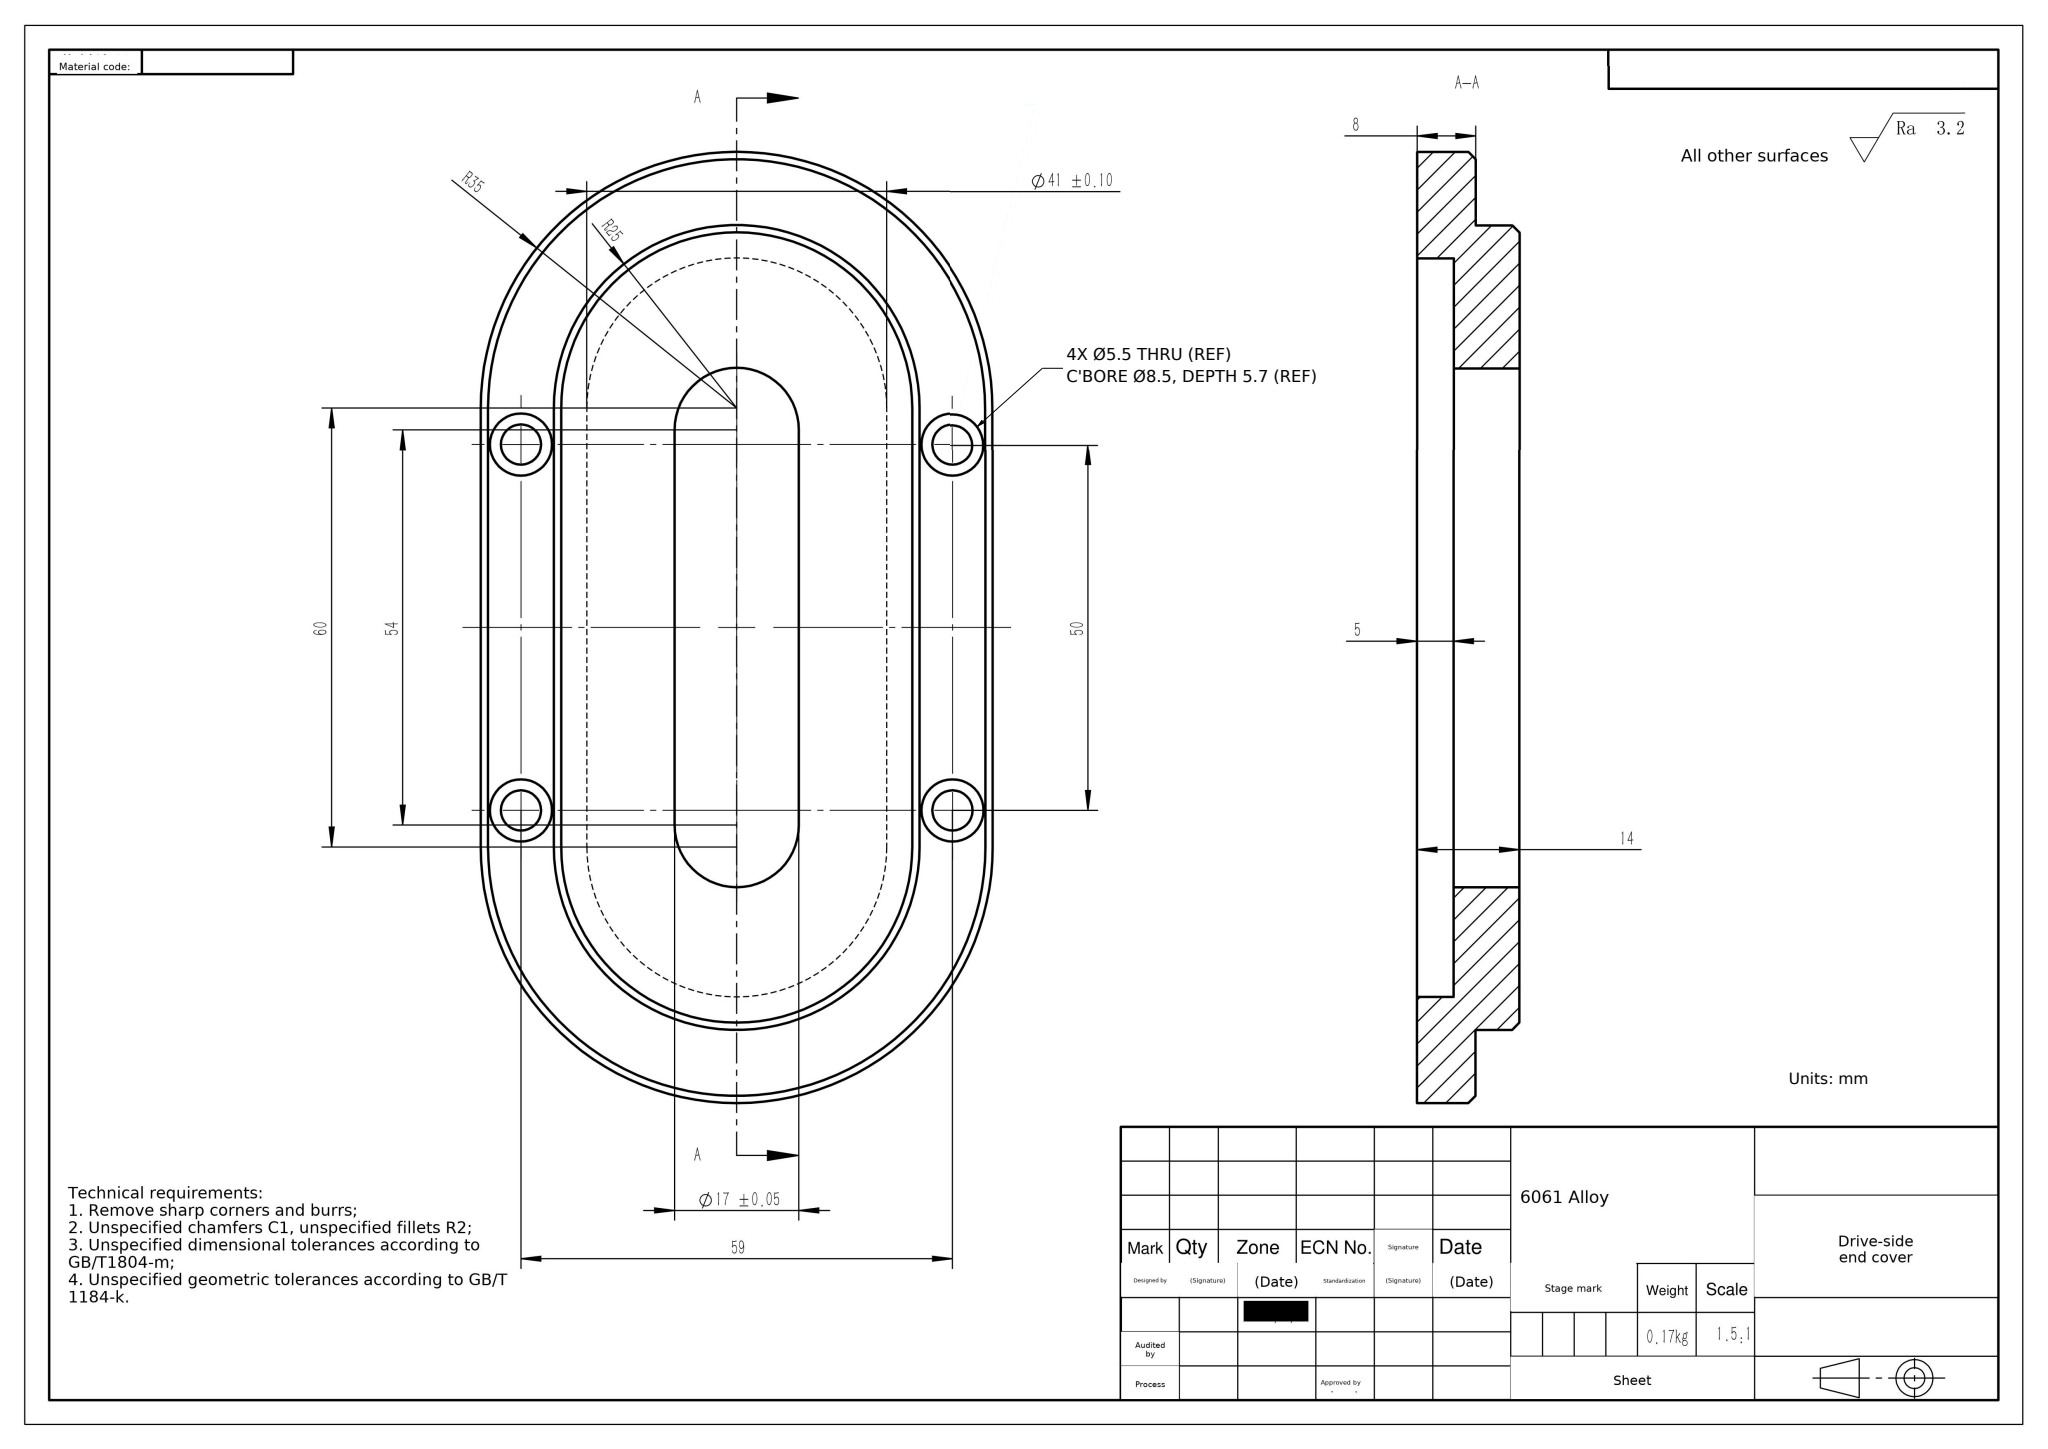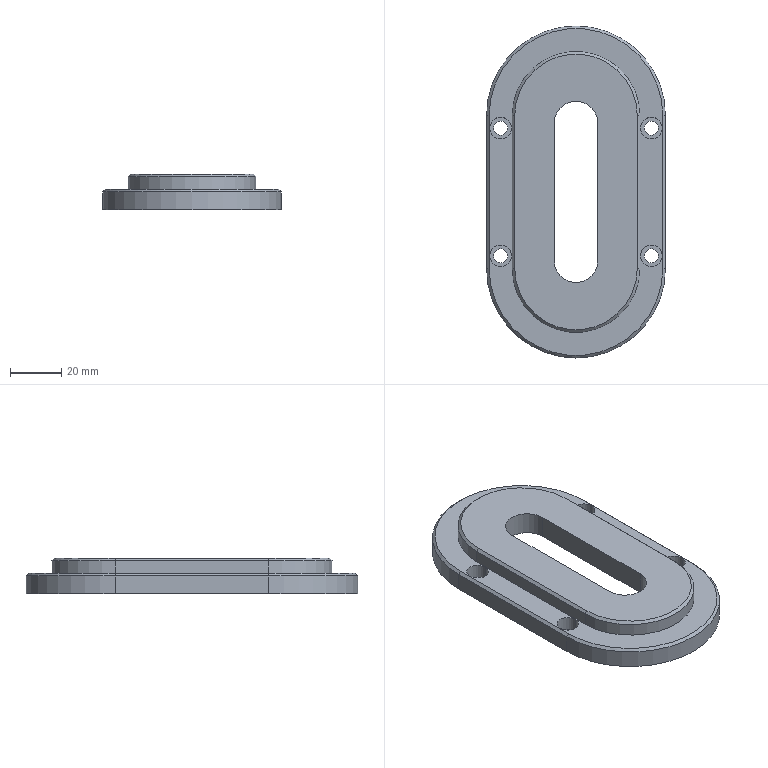Part | SolidWorks | mm | material 6061 Alloy | 1 solid | 48 faces | box 70 x 130 x 14 mm | volume 63144 mm3 | cylinder 24 | plane 20 | cone 4 | commonest cylinder face diameters 8.5 x8 5.5 x8 70 x2 41 x2 50 x2 17 x2
build123d program:
from build123d import *

# Parameters (mm, degrees)
BOSS_EXTRUDE1_DEPTH                             = 8
CUT_EXTRUDE1_DEPTH                              = 10
BOSS_EXTRUDE2_DEPTH                             = 6
CHAMFER1_SIZE                                   = 1
M5_HEX_SOCKET_HEAD_CAP_SCREW_CBORE1_D           = 5.5
M5_HEX_SOCKET_HEAD_CAP_SCREW_CBORE1_CBORE_D     = 8.5
M5_HEX_SOCKET_HEAD_CAP_SCREW_CBORE1_CBORE_DEPTH = 5.7
CUT_EXTRUDE2_DEPTH                              = 103.206
BOSS_EXTRUDE3_DEPTH                             = 3


with BuildPart() as part:
    # Sketch1 → Boss-Extrude1 (new body)
    with BuildSketch(Plane.XY):
        with BuildLine():
            Line((-35, 0), (-35, 60))
            ThreePointArc((-35, 60), (0, 95), (35, 60))
            Line((35, 60), (35, 0))
            ThreePointArc((35, 0), (0, -35), (-35, 0))
        make_face()
    extrude(amount=BOSS_EXTRUDE1_DEPTH)

    # Sketch2 → Cut-Extrude1 (cut)
    with BuildSketch(Plane(origin=(0, 0, 0), x_dir=(-1, 0, 0), z_dir=(0, 0, -1))):
        with BuildLine():
            Line((-20.5, 0), (-20.5, 60))
            ThreePointArc((-20.5, 60), (0, 80.5), (20.5, 60))
            Line((20.5, 60), (20.5, 0))
            ThreePointArc((20.5, 0), (0, -20.5), (-20.5, 0))
        make_face()
    extrude(amount=-CUT_EXTRUDE1_DEPTH, mode=Mode.SUBTRACT)

    # Sketch3 → Boss-Extrude2 (add)
    with BuildSketch(Plane.XY.offset(8)):
        with BuildLine():
            Line((25, 0), (25, 60))
            ThreePointArc((25, 60), (0, 85), (-25, 60))
            Line((-25, 60), (-25, 0))
            ThreePointArc((-25, 0), (0, -25), (25, 0))
        make_face()
    extrude(amount=BOSS_EXTRUDE2_DEPTH)

    # Chamfer1
    chamfer1_edges = [part.edges().sort_by_distance(p)[0] for p in [
        (0, 95, 8),
        (-35, 30, 8),
        (0, -25, 14),
        (25, 30, 14),
        (0, 85, 14),
        (-25, 30, 14),
        (0, -35, 8),
        (35, 30, 8),
    ]]
    chamfer(chamfer1_edges, length=CHAMFER1_SIZE)

    # M5 Hex Socket Head Cap Screw CBORE1 (through all)
    with Locations(Plane.XY.offset(8)):
        with Locations((-29.5, 55), (-29.5, 5), (29.5, 5), (29.5, 55)):
            CounterBoreHole(M5_HEX_SOCKET_HEAD_CAP_SCREW_CBORE1_D / 2, M5_HEX_SOCKET_HEAD_CAP_SCREW_CBORE1_CBORE_D / 2, M5_HEX_SOCKET_HEAD_CAP_SCREW_CBORE1_CBORE_DEPTH)

    # Sketch8 → Cut-Extrude2 (cut, through all)
    with BuildSketch(Plane.XY.offset(14)):
        with BuildLine():
            Line((-8.5, 3), (-8.5, 57))
            ThreePointArc((-8.5, 57), (0, 65.5), (8.5, 57))
            Line((8.5, 57), (8.5, 3))
            ThreePointArc((8.5, 3), (0, -5.5), (-8.5, 3))
        make_face()
    extrude(amount=-CUT_EXTRUDE2_DEPTH, mode=Mode.SUBTRACT)

    # Sketch9 → Boss-Extrude3 (add)
    with BuildSketch(Plane(origin=(0, 0, 8), x_dir=(-1, 0, 0), z_dir=(0, 0, -1))):
        with BuildLine():
            Line((-20.5, 60), (-20.5, 0))
            ThreePointArc((-20.5, 0), (0, -20.5), (20.5, 0))
            Line((20.5, 0), (20.5, 60))
            ThreePointArc((20.5, 60), (0, 80.5), (-20.5, 60))
        make_face()
        with BuildLine():
            Line((8.5, 57), (8.5, 3))
            ThreePointArc((8.5, 3), (0, -5.5), (-8.5, 3))
            Line((-8.5, 3), (-8.5, 57))
            ThreePointArc((-8.5, 57), (0, 65.5), (8.5, 57))
        make_face(mode=Mode.SUBTRACT)
    extrude(amount=BOSS_EXTRUDE3_DEPTH)


solid = part.part